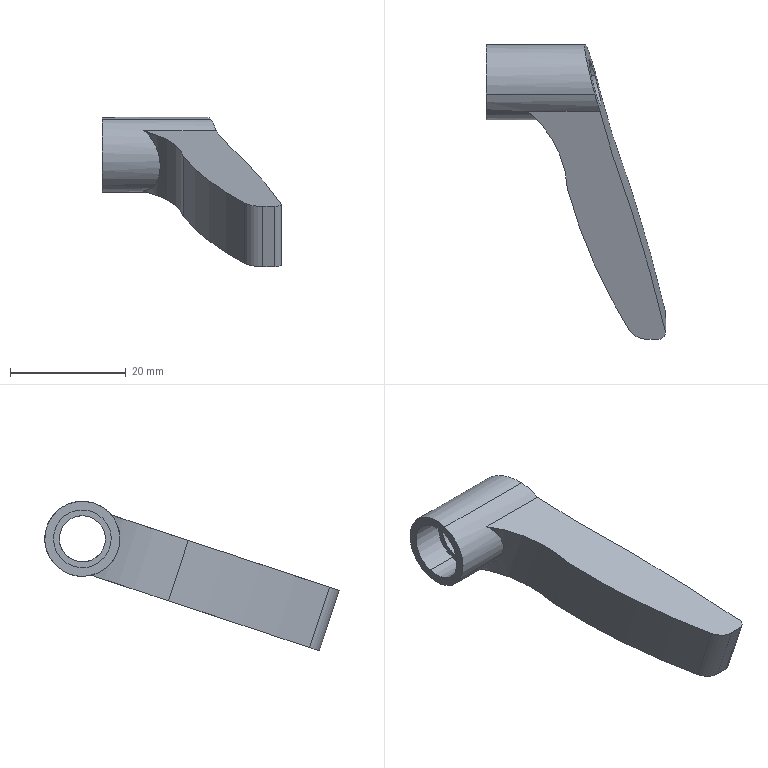Component | SolidWorks | SL010-LeftStreamline-1-1_SL010-2M-0112-000-2-1-1_SL010-CLDM5_25_B-1-1_SL010-_CLDM5_8_B_2_4-1-1 | 1 solid | 17 faces | box 31 x 50.95 x 25.87 mm | volume 5282 mm3 | cylinder 11 | plane 6 | commonest cylinder face diameters 13 x2 10 x2 8 x2 40 x1 200 x1 2.4 x1 600 x1 7.2 x1
STEP:
#1=COLOUR_RGB('',0.7922,0.8196,0.9333);
#2=FILL_AREA_STYLE_COLOUR('',#1);
#3=FILL_AREA_STYLE('',(#2));
#4=SURFACE_STYLE_FILL_AREA(#3);
#5=SURFACE_SIDE_STYLE('',(#4));
#6=SURFACE_STYLE_USAGE(.BOTH.,#5);
#7=PRESENTATION_STYLE_ASSIGNMENT((#6));
#8=CARTESIAN_POINT('',(-5.591,-6.762,-28.28));
#9=VERTEX_POINT('',#8);
#10=CARTESIAN_POINT('',(-5.859,-6.237,-28.106));
#11=VERTEX_POINT('',#10);
#12=CARTESIAN_POINT('',(-6.377,-6.8,-28.293));
#13=DIRECTION('',(0.,-0.3143,0.9493));
#14=DIRECTION('',(0.,-0.9493,-0.3143));
#15=AXIS2_PLACEMENT_3D('',#12,#13,#14);
#16=CIRCLE('',#15,0.7874);
#17=EDGE_CURVE('',#9,#11,#16,.T.);
#18=ORIENTED_EDGE('',*,*,#17,.T.);
#19=CARTESIAN_POINT('',(-5.859,-6.101,-28.518));
#20=VERTEX_POINT('',#19);
#21=CARTESIAN_POINT('',(-5.859,-6.101,-28.518));
#22=CARTESIAN_POINT('',(-5.842,-6.118,-28.513));
#23=CARTESIAN_POINT('',(-5.827,-6.135,-28.507));
#24=CARTESIAN_POINT('',(-5.807,-6.162,-28.494));
#25=CARTESIAN_POINT('',(-5.8,-6.171,-28.489));
#26=CARTESIAN_POINT('',(-5.788,-6.188,-28.478));
#27=CARTESIAN_POINT('',(-5.783,-6.197,-28.471));
#28=CARTESIAN_POINT('',(-5.773,-6.213,-28.457));
#29=CARTESIAN_POINT('',(-5.769,-6.221,-28.449));
#30=CARTESIAN_POINT('',(-5.761,-6.237,-28.432));
#31=CARTESIAN_POINT('',(-5.758,-6.244,-28.423));
#32=CARTESIAN_POINT('',(-5.753,-6.257,-28.404));
#33=CARTESIAN_POINT('',(-5.751,-6.263,-28.394));
#34=CARTESIAN_POINT('',(-5.749,-6.274,-28.372));
#35=CARTESIAN_POINT('',(-5.748,-6.279,-28.361));
#36=CARTESIAN_POINT('',(-5.748,-6.286,-28.339));
#37=CARTESIAN_POINT('',(-5.749,-6.289,-28.327));
#38=CARTESIAN_POINT('',(-5.751,-6.293,-28.303));
#39=CARTESIAN_POINT('',(-5.753,-6.295,-28.291));
#40=CARTESIAN_POINT('',(-5.758,-6.296,-28.268));
#41=CARTESIAN_POINT('',(-5.761,-6.295,-28.256));
#42=CARTESIAN_POINT('',(-5.769,-6.293,-28.234));
#43=CARTESIAN_POINT('',(-5.773,-6.291,-28.222));
#44=CARTESIAN_POINT('',(-5.783,-6.286,-28.201));
#45=CARTESIAN_POINT('',(-5.788,-6.283,-28.191));
#46=CARTESIAN_POINT('',(-5.8,-6.276,-28.171));
#47=CARTESIAN_POINT('',(-5.806,-6.272,-28.162));
#48=CARTESIAN_POINT('',(-5.827,-6.259,-28.135));
#49=CARTESIAN_POINT('',(-5.842,-6.248,-28.12));
#50=CARTESIAN_POINT('',(-5.859,-6.237,-28.106));
#51=B_SPLINE_CURVE_WITH_KNOTS('',3,(#21,#22,#23,#24,#25,#26,#27,#28,#29,#30,#31,#32,#33,#34,#35,#36,#37,#38,#39,#40,#41,#42,#43,#44,#45,#46,#47,#48,#49,#50),.UNSPECIFIED.,.F.,.F.,(4,2,2,2,2,2,2,2,2,2,2,2,2,2,4),(0.,0.00182,0.002729,0.003639,0.004549,0.005459,0.006368,0.007278,0.008188,0.009098,0.01001,0.01092,0.01183,0.01274,0.01456),.UNSPECIFIED.);
#52=EDGE_CURVE('',#20,#11,#51,.T.);
#53=ORIENTED_EDGE('',*,*,#52,.F.);
#54=CARTESIAN_POINT('',(-5.591,-6.626,-28.691));
#55=VERTEX_POINT('',#54);
#56=CARTESIAN_POINT('',(-6.377,-6.664,-28.704));
#57=DIRECTION('',(0.,-0.3143,0.9493));
#58=DIRECTION('',(0.,-0.9493,-0.3143));
#59=AXIS2_PLACEMENT_3D('',#56,#57,#58);
#60=CIRCLE('',#59,0.7874);
#61=EDGE_CURVE('',#55,#20,#60,.T.);
#62=ORIENTED_EDGE('',*,*,#61,.F.);
#63=CARTESIAN_POINT('',(-5.591,-6.762,-28.28));
#64=DIRECTION('',(-0.,0.3143,-0.9493));
#65=VECTOR('',#64,39.37);
#66=LINE('',#63,#65);
#67=EDGE_CURVE('',#9,#55,#66,.T.);
#68=ORIENTED_EDGE('',*,*,#67,.F.);
#69=EDGE_LOOP('',(#18,#53,#62,#68));
#70=FACE_OUTER_BOUND('',#69,.T.);
#71=CARTESIAN_POINT('',(-6.377,-6.8,-28.293));
#72=DIRECTION('',(0.,-0.3143,0.9493));
#73=DIRECTION('',(-0.8993,-0.4152,-0.1375));
#74=AXIS2_PLACEMENT_3D('',#71,#72,#73);
#75=CYLINDRICAL_SURFACE('',#74,0.7874);
#76=ADVANCED_FACE('',(#70),#75,.F.);
#77=CARTESIAN_POINT('',(-5.172,-7.587,-29.01));
#78=VERTEX_POINT('',#77);
#79=CARTESIAN_POINT('',(-1.778,-5.693,-28.382));
#80=DIRECTION('',(0.,-0.3143,0.9493));
#81=DIRECTION('',(0.,-0.9493,-0.3143));
#82=AXIS2_PLACEMENT_3D('',#79,#80,#81);
#83=CIRCLE('',#82,3.937);
#84=EDGE_CURVE('',#55,#78,#83,.T.);
#85=ORIENTED_EDGE('',*,*,#84,.T.);
#86=CARTESIAN_POINT('',(-5.172,-7.723,-28.598));
#87=VERTEX_POINT('',#86);
#88=CARTESIAN_POINT('',(-5.172,-7.723,-28.598));
#89=DIRECTION('',(-0.,0.3143,-0.9493));
#90=VECTOR('',#89,39.37);
#91=LINE('',#88,#90);
#92=EDGE_CURVE('',#87,#78,#91,.T.);
#93=ORIENTED_EDGE('',*,*,#92,.F.);
#94=CARTESIAN_POINT('',(-1.778,-5.829,-27.971));
#95=DIRECTION('',(0.,-0.3143,0.9493));
#96=DIRECTION('',(0.,-0.9493,-0.3143));
#97=AXIS2_PLACEMENT_3D('',#94,#95,#96);
#98=CIRCLE('',#97,3.937);
#99=EDGE_CURVE('',#9,#87,#98,.T.);
#100=ORIENTED_EDGE('',*,*,#99,.F.);
#101=ORIENTED_EDGE('',*,*,#67,.T.);
#102=EDGE_LOOP('',(#85,#93,#100,#101));
#103=FACE_OUTER_BOUND('',#102,.T.);
#104=CARTESIAN_POINT('',(-1.778,-5.829,-27.971));
#105=DIRECTION('',(0.,-0.3143,0.9493));
#106=DIRECTION('',(0.9242,0.3626,0.12));
#107=AXIS2_PLACEMENT_3D('',#104,#105,#106);
#108=CYLINDRICAL_SURFACE('',#107,3.937);
#109=ADVANCED_FACE('',(#103),#108,.T.);
#110=CARTESIAN_POINT('',(-4.921,-7.745,-28.606));
#111=VERTEX_POINT('',#110);
#112=CARTESIAN_POINT('',(-5.287,-6.522,-28.201));
#113=VERTEX_POINT('',#112);
#114=CARTESIAN_POINT('',(-16.448,-10.191,-29.416));
#115=DIRECTION('',(0.,-0.3143,0.9493));
#116=DIRECTION('',(0.,-0.9493,-0.3143));
#117=AXIS2_PLACEMENT_3D('',#114,#115,#116);
#118=CIRCLE('',#117,11.811);
#119=EDGE_CURVE('',#111,#113,#118,.T.);
#120=ORIENTED_EDGE('',*,*,#119,.T.);
#121=CARTESIAN_POINT('',(-5.367,-6.237,-28.106));
#122=VERTEX_POINT('',#121);
#123=CARTESIAN_POINT('',(-5.287,-6.523,-28.201));
#124=DIRECTION('',(-0.2588,0.917,0.3036));
#125=VECTOR('',#124,39.37);
#126=LINE('',#123,#125);
#127=EDGE_CURVE('',#113,#122,#126,.T.);
#128=ORIENTED_EDGE('',*,*,#127,.T.);
#129=CARTESIAN_POINT('',(-6.142,-6.237,-28.106));
#130=DIRECTION('',(-1.,-0.,0.));
#131=VECTOR('',#130,39.37);
#132=LINE('',#129,#131);
#133=EDGE_CURVE('',#122,#11,#132,.T.);
#134=ORIENTED_EDGE('',*,*,#133,.T.);
#135=ORIENTED_EDGE('',*,*,#17,.F.);
#136=ORIENTED_EDGE('',*,*,#99,.T.);
#137=CARTESIAN_POINT('',(-5.05,-7.789,-28.62));
#138=VERTEX_POINT('',#137);
#139=CARTESIAN_POINT('',(-5.05,-7.655,-28.576));
#140=DIRECTION('',(0.,-0.3143,0.9493));
#141=DIRECTION('',(0.,-0.9493,-0.3143));
#142=AXIS2_PLACEMENT_3D('',#139,#140,#141);
#143=CIRCLE('',#142,0.1417);
#144=EDGE_CURVE('',#87,#138,#143,.T.);
#145=ORIENTED_EDGE('',*,*,#144,.T.);
#146=CARTESIAN_POINT('',(-4.969,-7.789,-28.62));
#147=VERTEX_POINT('',#146);
#148=CARTESIAN_POINT('',(-5.05,-7.789,-28.62));
#149=DIRECTION('',(1.,0.,-0.));
#150=VECTOR('',#149,39.37);
#151=LINE('',#148,#150);
#152=EDGE_CURVE('',#138,#147,#151,.T.);
#153=ORIENTED_EDGE('',*,*,#152,.T.);
#154=CARTESIAN_POINT('',(-4.969,-7.745,-28.606));
#155=DIRECTION('',(0.,-0.3143,0.9493));
#156=DIRECTION('',(0.,-0.9493,-0.3143));
#157=AXIS2_PLACEMENT_3D('',#154,#155,#156);
#158=CIRCLE('',#157,0.04724);
#159=EDGE_CURVE('',#147,#111,#158,.T.);
#160=ORIENTED_EDGE('',*,*,#159,.T.);
#161=EDGE_LOOP('',(#120,#128,#134,#135,#136,#145,#153,#160));
#162=FACE_OUTER_BOUND('',#161,.T.);
#163=CARTESIAN_POINT('',(-6.377,-6.8,-28.293));
#164=DIRECTION('',(0.,-0.3143,0.9493));
#165=DIRECTION('',(0.,-0.9493,-0.3143));
#166=AXIS2_PLACEMENT_3D('',#163,#164,#165);
#167=PLANE('',#166);
#168=ADVANCED_FACE('',(#162),#167,.T.);
#169=ORIENTED_EDGE('',*,*,#159,.F.);
#170=CARTESIAN_POINT('',(-4.969,-7.653,-29.032));
#171=VERTEX_POINT('',#170);
#172=CARTESIAN_POINT('',(-4.969,-7.814,-28.546));
#173=DIRECTION('',(-0.,0.3143,-0.9493));
#174=VECTOR('',#173,39.37);
#175=LINE('',#172,#174);
#176=EDGE_CURVE('',#147,#171,#175,.T.);
#177=ORIENTED_EDGE('',*,*,#176,.T.);
#178=CARTESIAN_POINT('',(-4.921,-7.608,-29.017));
#179=VERTEX_POINT('',#178);
#180=CARTESIAN_POINT('',(-4.969,-7.608,-29.017));
#181=DIRECTION('',(0.,-0.3143,0.9493));
#182=DIRECTION('',(0.,-0.9493,-0.3143));
#183=AXIS2_PLACEMENT_3D('',#180,#181,#182);
#184=CIRCLE('',#183,0.04724);
#185=EDGE_CURVE('',#171,#179,#184,.T.);
#186=ORIENTED_EDGE('',*,*,#185,.T.);
#187=CARTESIAN_POINT('',(-4.921,-7.769,-28.531));
#188=DIRECTION('',(-0.,0.3143,-0.9493));
#189=VECTOR('',#188,39.37);
#190=LINE('',#187,#189);
#191=EDGE_CURVE('',#111,#179,#190,.T.);
#192=ORIENTED_EDGE('',*,*,#191,.F.);
#193=EDGE_LOOP('',(#169,#177,#186,#192));
#194=FACE_OUTER_BOUND('',#193,.T.);
#195=CARTESIAN_POINT('',(-4.969,-7.769,-28.531));
#196=DIRECTION('',(0.,-0.3143,0.9493));
#197=DIRECTION('',(-0.7071,0.6713,0.2223));
#198=AXIS2_PLACEMENT_3D('',#195,#196,#197);
#199=CYLINDRICAL_SURFACE('',#198,0.04724);
#200=ADVANCED_FACE('',(#194),#199,.T.);
#201=ORIENTED_EDGE('',*,*,#119,.F.);
#202=ORIENTED_EDGE('',*,*,#191,.T.);
#203=CARTESIAN_POINT('',(-5.287,-6.386,-28.612));
#204=VERTEX_POINT('',#203);
#205=CARTESIAN_POINT('',(-16.448,-10.055,-29.827));
#206=DIRECTION('',(0.,-0.3143,0.9493));
#207=DIRECTION('',(0.,-0.9493,-0.3143));
#208=AXIS2_PLACEMENT_3D('',#205,#206,#207);
#209=CIRCLE('',#208,11.811);
#210=EDGE_CURVE('',#179,#204,#209,.T.);
#211=ORIENTED_EDGE('',*,*,#210,.T.);
#212=CARTESIAN_POINT('',(-5.287,-6.547,-28.126));
#213=DIRECTION('',(-0.,0.3143,-0.9493));
#214=VECTOR('',#213,39.37);
#215=LINE('',#212,#214);
#216=EDGE_CURVE('',#113,#204,#215,.T.);
#217=ORIENTED_EDGE('',*,*,#216,.F.);
#218=EDGE_LOOP('',(#201,#202,#211,#217));
#219=FACE_OUTER_BOUND('',#218,.T.);
#220=CARTESIAN_POINT('',(-16.448,-10.216,-29.341));
#221=DIRECTION('',(0.,-0.3143,0.9493));
#222=DIRECTION('',(-0.962,-0.2593,-0.08585));
#223=AXIS2_PLACEMENT_3D('',#220,#221,#222);
#224=CYLINDRICAL_SURFACE('',#223,11.811);
#225=ADVANCED_FACE('',(#219),#224,.T.);
#226=CARTESIAN_POINT('',(-5.362,-6.189,-28.319));
#227=VERTEX_POINT('',#226);
#228=CARTESIAN_POINT('',(-5.404,-5.99,-28.419));
#229=VERTEX_POINT('',#228);
#230=CARTESIAN_POINT('',(-5.362,-6.189,-28.319));
#231=CARTESIAN_POINT('',(-5.362,-6.183,-28.338));
#232=CARTESIAN_POINT('',(-5.363,-6.172,-28.356));
#233=CARTESIAN_POINT('',(-5.367,-6.145,-28.388));
#234=CARTESIAN_POINT('',(-5.37,-6.129,-28.401));
#235=CARTESIAN_POINT('',(-5.378,-6.092,-28.419));
#236=CARTESIAN_POINT('',(-5.383,-6.072,-28.425));
#237=CARTESIAN_POINT('',(-5.393,-6.03,-28.428));
#238=CARTESIAN_POINT('',(-5.398,-6.01,-28.425));
#239=CARTESIAN_POINT('',(-5.404,-5.99,-28.419));
#240=B_SPLINE_CURVE_WITH_KNOTS('',3,(#230,#231,#232,#233,#234,#235,#236,#237,#238,#239),.UNSPECIFIED.,.F.,.F.,(4,2,2,2,4),(0.,0.3927,0.7854,1.178,1.571),.UNSPECIFIED.);
#241=EDGE_CURVE('',#227,#229,#240,.T.);
#242=ORIENTED_EDGE('',*,*,#241,.F.);
#243=CARTESIAN_POINT('',(-5.404,-6.089,-28.12));
#244=VERTEX_POINT('',#243);
#245=CARTESIAN_POINT('',(-5.404,-6.089,-28.12));
#246=CARTESIAN_POINT('',(-5.398,-6.109,-28.126));
#247=CARTESIAN_POINT('',(-5.393,-6.127,-28.136));
#248=CARTESIAN_POINT('',(-5.383,-6.158,-28.163));
#249=CARTESIAN_POINT('',(-5.378,-6.171,-28.18));
#250=CARTESIAN_POINT('',(-5.37,-6.19,-28.217));
#251=CARTESIAN_POINT('',(-5.367,-6.195,-28.237));
#252=CARTESIAN_POINT('',(-5.363,-6.198,-28.278));
#253=CARTESIAN_POINT('',(-5.362,-6.196,-28.299));
#254=CARTESIAN_POINT('',(-5.362,-6.189,-28.319));
#255=B_SPLINE_CURVE_WITH_KNOTS('',3,(#245,#246,#247,#248,#249,#250,#251,#252,#253,#254),.UNSPECIFIED.,.F.,.F.,(4,2,2,2,4),(4.712,5.105,5.498,5.89,6.283),.UNSPECIFIED.);
#256=EDGE_CURVE('',#244,#227,#255,.T.);
#257=ORIENTED_EDGE('',*,*,#256,.F.);
#258=CARTESIAN_POINT('',(-5.404,-5.99,-28.419));
#259=CARTESIAN_POINT('',(-5.409,-5.97,-28.412));
#260=CARTESIAN_POINT('',(-5.415,-5.952,-28.402));
#261=CARTESIAN_POINT('',(-5.425,-5.921,-28.375));
#262=CARTESIAN_POINT('',(-5.43,-5.908,-28.358));
#263=CARTESIAN_POINT('',(-5.438,-5.89,-28.321));
#264=CARTESIAN_POINT('',(-5.441,-5.884,-28.301));
#265=CARTESIAN_POINT('',(-5.445,-5.881,-28.26));
#266=CARTESIAN_POINT('',(-5.446,-5.884,-28.239));
#267=CARTESIAN_POINT('',(-5.446,-5.897,-28.2));
#268=CARTESIAN_POINT('',(-5.445,-5.907,-28.182));
#269=CARTESIAN_POINT('',(-5.441,-5.934,-28.151));
#270=CARTESIAN_POINT('',(-5.438,-5.95,-28.138));
#271=CARTESIAN_POINT('',(-5.43,-5.987,-28.119));
#272=CARTESIAN_POINT('',(-5.425,-6.007,-28.114));
#273=CARTESIAN_POINT('',(-5.415,-6.049,-28.111));
#274=CARTESIAN_POINT('',(-5.409,-6.069,-28.113));
#275=CARTESIAN_POINT('',(-5.404,-6.089,-28.12));
#276=B_SPLINE_CURVE_WITH_KNOTS('',3,(#258,#259,#260,#261,#262,#263,#264,#265,#266,#267,#268,#269,#270,#271,#272,#273,#274,#275),.UNSPECIFIED.,.F.,.F.,(4,2,2,2,2,2,2,2,4),(1.571,1.963,2.356,2.749,3.142,3.534,3.927,4.32,4.712),.UNSPECIFIED.);
#277=EDGE_CURVE('',#229,#244,#276,.T.);
#278=ORIENTED_EDGE('',*,*,#277,.F.);
#279=EDGE_LOOP('',(#242,#257,#278));
#280=FACE_BOUND('',#279,.T.);
#281=ORIENTED_EDGE('',*,*,#216,.T.);
#282=CARTESIAN_POINT('',(-5.367,-6.101,-28.518));
#283=VERTEX_POINT('',#282);
#284=CARTESIAN_POINT('',(-5.287,-6.387,-28.612));
#285=DIRECTION('',(-0.2588,0.917,0.3036));
#286=VECTOR('',#285,39.37);
#287=LINE('',#284,#286);
#288=EDGE_CURVE('',#204,#283,#287,.T.);
#289=ORIENTED_EDGE('',*,*,#288,.T.);
#290=CARTESIAN_POINT('',(-5.404,-5.959,-28.512));
#291=VERTEX_POINT('',#290);
#292=CARTESIAN_POINT('',(-5.367,-6.101,-28.518));
#293=CARTESIAN_POINT('',(-5.373,-6.078,-28.523));
#294=CARTESIAN_POINT('',(-5.379,-6.054,-28.526));
#295=CARTESIAN_POINT('',(-5.391,-6.006,-28.524));
#296=CARTESIAN_POINT('',(-5.398,-5.982,-28.519));
#297=CARTESIAN_POINT('',(-5.404,-5.959,-28.512));
#298=B_SPLINE_CURVE_WITH_KNOTS('',3,(#292,#293,#294,#295,#296,#297),.UNSPECIFIED.,.F.,.F.,(4,2,4),(0.,1.5,3.),.UNSPECIFIED.);
#299=EDGE_CURVE('',#283,#291,#298,.T.);
#300=ORIENTED_EDGE('',*,*,#299,.T.);
#301=CARTESIAN_POINT('',(-5.404,-6.12,-28.026));
#302=VERTEX_POINT('',#301);
#303=CARTESIAN_POINT('',(-5.404,-5.959,-28.512));
#304=CARTESIAN_POINT('',(-5.408,-5.945,-28.507));
#305=CARTESIAN_POINT('',(-5.412,-5.93,-28.501));
#306=CARTESIAN_POINT('',(-5.421,-5.902,-28.486));
#307=CARTESIAN_POINT('',(-5.425,-5.888,-28.476));
#308=CARTESIAN_POINT('',(-5.433,-5.862,-28.455));
#309=CARTESIAN_POINT('',(-5.437,-5.85,-28.442));
#310=CARTESIAN_POINT('',(-5.445,-5.828,-28.415));
#311=CARTESIAN_POINT('',(-5.449,-5.819,-28.4));
#312=CARTESIAN_POINT('',(-5.456,-5.803,-28.368));
#313=CARTESIAN_POINT('',(-5.459,-5.797,-28.352));
#314=CARTESIAN_POINT('',(-5.464,-5.788,-28.318));
#315=CARTESIAN_POINT('',(-5.466,-5.785,-28.301));
#316=CARTESIAN_POINT('',(-5.469,-5.783,-28.267));
#317=CARTESIAN_POINT('',(-5.471,-5.784,-28.25));
#318=CARTESIAN_POINT('',(-5.472,-5.788,-28.218));
#319=CARTESIAN_POINT('',(-5.472,-5.792,-28.203));
#320=CARTESIAN_POINT('',(-5.472,-5.801,-28.174));
#321=CARTESIAN_POINT('',(-5.472,-5.808,-28.16));
#322=CARTESIAN_POINT('',(-5.471,-5.823,-28.132));
#323=CARTESIAN_POINT('',(-5.469,-5.832,-28.118));
#324=CARTESIAN_POINT('',(-5.466,-5.854,-28.092));
#325=CARTESIAN_POINT('',(-5.464,-5.867,-28.08));
#326=CARTESIAN_POINT('',(-5.459,-5.894,-28.058));
#327=CARTESIAN_POINT('',(-5.456,-5.909,-28.048));
#328=CARTESIAN_POINT('',(-5.449,-5.94,-28.033));
#329=CARTESIAN_POINT('',(-5.445,-5.957,-28.026));
#330=CARTESIAN_POINT('',(-5.437,-5.991,-28.017));
#331=CARTESIAN_POINT('',(-5.433,-6.008,-28.015));
#332=CARTESIAN_POINT('',(-5.425,-6.042,-28.013));
#333=CARTESIAN_POINT('',(-5.421,-6.058,-28.013));
#334=CARTESIAN_POINT('',(-5.412,-6.09,-28.018));
#335=CARTESIAN_POINT('',(-5.408,-6.106,-28.021));
#336=CARTESIAN_POINT('',(-5.404,-6.12,-28.026));
#337=B_SPLINE_CURVE_WITH_KNOTS('',3,(#303,#304,#305,#306,#307,#308,#309,#310,#311,#312,#313,#314,#315,#316,#317,#318,#319,#320,#321,#322,#323,#324,#325,#326,#327,#328,#329,#330,#331,#332,#333,#334,#335,#336),.UNSPECIFIED.,.F.,.F.,(4,2,2,2,2,2,2,2,2,2,2,2,2,2,2,2,4),(0.,0.0625,0.125,0.1875,0.25,0.3125,0.375,0.4375,0.5,0.5625,0.625,0.6875,0.75,0.8125,0.875,0.9375,1.),.UNSPECIFIED.);
#338=EDGE_CURVE('',#291,#302,#337,.T.);
#339=ORIENTED_EDGE('',*,*,#338,.T.);
#340=CARTESIAN_POINT('',(-5.404,-6.12,-28.026));
#341=CARTESIAN_POINT('',(-5.398,-6.142,-28.034));
#342=CARTESIAN_POINT('',(-5.391,-6.164,-28.044));
#343=CARTESIAN_POINT('',(-5.379,-6.204,-28.072));
#344=CARTESIAN_POINT('',(-5.373,-6.222,-28.088));
#345=CARTESIAN_POINT('',(-5.367,-6.237,-28.106));
#346=B_SPLINE_CURVE_WITH_KNOTS('',3,(#340,#341,#342,#343,#344,#345),.UNSPECIFIED.,.F.,.F.,(4,2,4),(0.,1.5,3.),.UNSPECIFIED.);
#347=EDGE_CURVE('',#302,#122,#346,.T.);
#348=ORIENTED_EDGE('',*,*,#347,.T.);
#349=ORIENTED_EDGE('',*,*,#127,.F.);
#350=EDGE_LOOP('',(#281,#289,#300,#339,#348,#349));
#351=FACE_OUTER_BOUND('',#350,.T.);
#352=CARTESIAN_POINT('',(-5.472,-5.889,-27.908));
#353=DIRECTION('',(0.9659,0.2457,0.08135));
#354=DIRECTION('',(-0.2588,0.917,0.3036));
#355=AXIS2_PLACEMENT_3D('',#352,#353,#354);
#356=PLANE('',#355);
#357=ADVANCED_FACE('',(#280,#351),#356,.T.);
#358=CARTESIAN_POINT('',(-6.142,-5.959,-28.512));
#359=VERTEX_POINT('',#358);
#360=CARTESIAN_POINT('',(-6.142,-6.12,-28.026));
#361=VERTEX_POINT('',#360);
#362=CARTESIAN_POINT('',(-6.142,-6.04,-28.269));
#363=DIRECTION('',(-1.,-0.,0.));
#364=DIRECTION('',(0.,0.3143,-0.9493));
#365=AXIS2_PLACEMENT_3D('',#362,#363,#364);
#366=CIRCLE('',#365,0.2559);
#367=EDGE_CURVE('',#359,#361,#366,.T.);
#368=ORIENTED_EDGE('',*,*,#367,.F.);
#369=CARTESIAN_POINT('',(-6.142,-5.959,-28.512));
#370=DIRECTION('',(1.,0.,-0.));
#371=VECTOR('',#370,39.37);
#372=LINE('',#369,#371);
#373=EDGE_CURVE('',#359,#291,#372,.T.);
#374=ORIENTED_EDGE('',*,*,#373,.T.);
#375=ORIENTED_EDGE('',*,*,#299,.F.);
#376=CARTESIAN_POINT('',(-6.142,-6.101,-28.518));
#377=DIRECTION('',(-1.,-0.,0.));
#378=VECTOR('',#377,39.37);
#379=LINE('',#376,#378);
#380=EDGE_CURVE('',#283,#20,#379,.T.);
#381=ORIENTED_EDGE('',*,*,#380,.T.);
#382=ORIENTED_EDGE('',*,*,#52,.T.);
#383=ORIENTED_EDGE('',*,*,#133,.F.);
#384=ORIENTED_EDGE('',*,*,#347,.F.);
#385=CARTESIAN_POINT('',(-6.142,-6.12,-28.026));
#386=DIRECTION('',(1.,0.,-0.));
#387=VECTOR('',#386,39.37);
#388=LINE('',#385,#387);
#389=EDGE_CURVE('',#361,#302,#388,.T.);
#390=ORIENTED_EDGE('',*,*,#389,.F.);
#391=EDGE_LOOP('',(#368,#374,#375,#381,#382,#383,#384,#390));
#392=FACE_OUTER_BOUND('',#391,.T.);
#393=CARTESIAN_POINT('',(-6.142,-6.04,-28.269));
#394=DIRECTION('',(1.,0.,-0.));
#395=DIRECTION('',(0.,0.9493,0.3143));
#396=AXIS2_PLACEMENT_3D('',#393,#394,#395);
#397=CYLINDRICAL_SURFACE('',#396,0.2559);
#398=ADVANCED_FACE('',(#392),#397,.T.);
#399=ORIENTED_EDGE('',*,*,#338,.F.);
#400=ORIENTED_EDGE('',*,*,#373,.F.);
#401=CARTESIAN_POINT('',(-6.142,-6.04,-28.269));
#402=DIRECTION('',(-1.,-0.,0.));
#403=DIRECTION('',(0.,0.3143,-0.9493));
#404=AXIS2_PLACEMENT_3D('',#401,#402,#403);
#405=CIRCLE('',#404,0.2559);
#406=EDGE_CURVE('',#361,#359,#405,.T.);
#407=ORIENTED_EDGE('',*,*,#406,.F.);
#408=ORIENTED_EDGE('',*,*,#389,.T.);
#409=EDGE_LOOP('',(#399,#400,#407,#408));
#410=FACE_OUTER_BOUND('',#409,.T.);
#411=CARTESIAN_POINT('',(-6.142,-6.04,-28.269));
#412=DIRECTION('',(1.,0.,-0.));
#413=DIRECTION('',(0.,-0.9493,-0.3143));
#414=AXIS2_PLACEMENT_3D('',#411,#412,#413);
#415=CYLINDRICAL_SURFACE('',#414,0.2559);
#416=ADVANCED_FACE('',(#410),#415,.T.);
#417=CARTESIAN_POINT('',(-6.142,-6.101,-28.082));
#418=VERTEX_POINT('',#417);
#419=CARTESIAN_POINT('',(-6.142,-5.978,-28.456));
#420=VERTEX_POINT('',#419);
#421=CARTESIAN_POINT('',(-6.142,-6.04,-28.269));
#422=DIRECTION('',(1.,0.,-0.));
#423=DIRECTION('',(0.,-0.3143,0.9493));
#424=AXIS2_PLACEMENT_3D('',#421,#422,#423);
#425=CIRCLE('',#424,0.1969);
#426=EDGE_CURVE('',#418,#420,#425,.T.);
#427=ORIENTED_EDGE('',*,*,#426,.T.);
#428=CARTESIAN_POINT('',(-6.142,-6.04,-28.269));
#429=DIRECTION('',(1.,0.,-0.));
#430=DIRECTION('',(0.,-0.3143,0.9493));
#431=AXIS2_PLACEMENT_3D('',#428,#429,#430);
#432=CIRCLE('',#431,0.1969);
#433=EDGE_CURVE('',#420,#418,#432,.T.);
#434=ORIENTED_EDGE('',*,*,#433,.T.);
#435=EDGE_LOOP('',(#427,#434));
#436=FACE_BOUND('',#435,.T.);
#437=ORIENTED_EDGE('',*,*,#367,.T.);
#438=ORIENTED_EDGE('',*,*,#406,.T.);
#439=EDGE_LOOP('',(#437,#438));
#440=FACE_OUTER_BOUND('',#439,.T.);
#441=CARTESIAN_POINT('',(-6.142,-6.282,-28.35));
#442=DIRECTION('',(1.,0.,-0.));
#443=DIRECTION('',(0.,-0.3143,0.9493));
#444=AXIS2_PLACEMENT_3D('',#441,#442,#443);
#445=PLANE('',#444);
#446=ADVANCED_FACE('',(#436,#440),#445,.F.);
#447=ORIENTED_EDGE('',*,*,#433,.F.);
#448=CARTESIAN_POINT('',(-5.929,-5.978,-28.456));
#449=VERTEX_POINT('',#448);
#450=CARTESIAN_POINT('',(-5.929,-5.978,-28.456));
#451=DIRECTION('',(-1.,-0.,0.));
#452=VECTOR('',#451,39.37);
#453=LINE('',#450,#452);
#454=EDGE_CURVE('',#449,#420,#453,.T.);
#455=ORIENTED_EDGE('',*,*,#454,.F.);
#456=CARTESIAN_POINT('',(-5.929,-6.101,-28.082));
#457=VERTEX_POINT('',#456);
#458=CARTESIAN_POINT('',(-5.929,-6.04,-28.269));
#459=DIRECTION('',(1.,0.,-0.));
#460=DIRECTION('',(0.,-0.3143,0.9493));
#461=AXIS2_PLACEMENT_3D('',#458,#459,#460);
#462=CIRCLE('',#461,0.1969);
#463=EDGE_CURVE('',#449,#457,#462,.T.);
#464=ORIENTED_EDGE('',*,*,#463,.T.);
#465=CARTESIAN_POINT('',(-5.929,-6.101,-28.082));
#466=DIRECTION('',(-1.,-0.,0.));
#467=VECTOR('',#466,39.37);
#468=LINE('',#465,#467);
#469=EDGE_CURVE('',#457,#418,#468,.T.);
#470=ORIENTED_EDGE('',*,*,#469,.T.);
#471=EDGE_LOOP('',(#447,#455,#464,#470));
#472=FACE_OUTER_BOUND('',#471,.T.);
#473=CARTESIAN_POINT('',(-4.331,-6.04,-28.269));
#474=DIRECTION('',(-1.,-0.,0.));
#475=DIRECTION('',(0.,-0.9493,-0.3143));
#476=AXIS2_PLACEMENT_3D('',#473,#474,#475);
#477=CYLINDRICAL_SURFACE('',#476,0.1969);
#478=ADVANCED_FACE('',(#472),#477,.F.);
#479=CARTESIAN_POINT('',(-5.929,-6.04,-28.269));
#480=DIRECTION('',(1.,0.,-0.));
#481=DIRECTION('',(0.,-0.3143,0.9493));
#482=AXIS2_PLACEMENT_3D('',#479,#480,#481);
#483=CIRCLE('',#482,0.1969);
#484=EDGE_CURVE('',#457,#449,#483,.T.);
#485=ORIENTED_EDGE('',*,*,#484,.T.);
#486=ORIENTED_EDGE('',*,*,#454,.T.);
#487=ORIENTED_EDGE('',*,*,#426,.F.);
#488=ORIENTED_EDGE('',*,*,#469,.F.);
#489=EDGE_LOOP('',(#485,#486,#487,#488));
#490=FACE_OUTER_BOUND('',#489,.T.);
#491=CARTESIAN_POINT('',(-4.331,-6.04,-28.269));
#492=DIRECTION('',(-1.,-0.,0.));
#493=DIRECTION('',(0.,0.9493,0.3143));
#494=AXIS2_PLACEMENT_3D('',#491,#492,#493);
#495=CYLINDRICAL_SURFACE('',#494,0.1969);
#496=ADVANCED_FACE('',(#490),#495,.F.);
#497=CARTESIAN_POINT('',(-5.929,-6.089,-28.12));
#498=VERTEX_POINT('',#497);
#499=CARTESIAN_POINT('',(-5.929,-5.99,-28.419));
#500=VERTEX_POINT('',#499);
#501=CARTESIAN_POINT('',(-5.929,-6.04,-28.269));
#502=DIRECTION('',(1.,0.,-0.));
#503=DIRECTION('',(0.,-0.3143,0.9493));
#504=AXIS2_PLACEMENT_3D('',#501,#502,#503);
#505=CIRCLE('',#504,0.1575);
#506=EDGE_CURVE('',#498,#500,#505,.T.);
#507=ORIENTED_EDGE('',*,*,#506,.T.);
#508=CARTESIAN_POINT('',(-5.929,-6.04,-28.269));
#509=DIRECTION('',(1.,0.,-0.));
#510=DIRECTION('',(0.,-0.3143,0.9493));
#511=AXIS2_PLACEMENT_3D('',#508,#509,#510);
#512=CIRCLE('',#511,0.1575);
#513=EDGE_CURVE('',#500,#498,#512,.T.);
#514=ORIENTED_EDGE('',*,*,#513,.T.);
#515=EDGE_LOOP('',(#507,#514));
#516=FACE_BOUND('',#515,.T.);
#517=ORIENTED_EDGE('',*,*,#484,.F.);
#518=ORIENTED_EDGE('',*,*,#463,.F.);
#519=EDGE_LOOP('',(#517,#518));
#520=FACE_OUTER_BOUND('',#519,.T.);
#521=CARTESIAN_POINT('',(-5.929,-5.853,-28.207));
#522=DIRECTION('',(-1.,-0.,0.));
#523=DIRECTION('',(-0.,0.3143,-0.9493));
#524=AXIS2_PLACEMENT_3D('',#521,#522,#523);
#525=PLANE('',#524);
#526=ADVANCED_FACE('',(#516,#520),#525,.T.);
#527=ORIENTED_EDGE('',*,*,#513,.F.);
#528=CARTESIAN_POINT('',(-5.404,-5.99,-28.419));
#529=DIRECTION('',(-1.,-0.,0.));
#530=VECTOR('',#529,39.37);
#531=LINE('',#528,#530);
#532=EDGE_CURVE('',#229,#500,#531,.T.);
#533=ORIENTED_EDGE('',*,*,#532,.F.);
#534=ORIENTED_EDGE('',*,*,#277,.T.);
#535=CARTESIAN_POINT('',(-5.404,-6.089,-28.12));
#536=DIRECTION('',(-1.,-0.,0.));
#537=VECTOR('',#536,39.37);
#538=LINE('',#535,#537);
#539=EDGE_CURVE('',#244,#498,#538,.T.);
#540=ORIENTED_EDGE('',*,*,#539,.T.);
#541=EDGE_LOOP('',(#527,#533,#534,#540));
#542=FACE_OUTER_BOUND('',#541,.T.);
#543=CARTESIAN_POINT('',(-4.331,-6.04,-28.269));
#544=DIRECTION('',(-1.,-0.,0.));
#545=DIRECTION('',(0.,-0.9493,-0.3143));
#546=AXIS2_PLACEMENT_3D('',#543,#544,#545);
#547=CYLINDRICAL_SURFACE('',#546,0.1575);
#548=ADVANCED_FACE('',(#542),#547,.F.);
#549=ORIENTED_EDGE('',*,*,#241,.T.);
#550=ORIENTED_EDGE('',*,*,#532,.T.);
#551=ORIENTED_EDGE('',*,*,#506,.F.);
#552=ORIENTED_EDGE('',*,*,#539,.F.);
#553=ORIENTED_EDGE('',*,*,#256,.T.);
#554=EDGE_LOOP('',(#549,#550,#551,#552,#553));
#555=FACE_OUTER_BOUND('',#554,.T.);
#556=CARTESIAN_POINT('',(-4.331,-6.04,-28.269));
#557=DIRECTION('',(-1.,-0.,0.));
#558=DIRECTION('',(0.,0.9493,0.3143));
#559=AXIS2_PLACEMENT_3D('',#556,#557,#558);
#560=CYLINDRICAL_SURFACE('',#559,0.1575);
#561=ADVANCED_FACE('',(#555),#560,.F.);
#562=ORIENTED_EDGE('',*,*,#288,.F.);
#563=ORIENTED_EDGE('',*,*,#210,.F.);
#564=ORIENTED_EDGE('',*,*,#185,.F.);
#565=CARTESIAN_POINT('',(-5.05,-7.653,-29.032));
#566=VERTEX_POINT('',#565);
#567=CARTESIAN_POINT('',(-5.05,-7.653,-29.032));
#568=DIRECTION('',(1.,0.,-0.));
#569=VECTOR('',#568,39.37);
#570=LINE('',#567,#569);
#571=EDGE_CURVE('',#566,#171,#570,.T.);
#572=ORIENTED_EDGE('',*,*,#571,.F.);
#573=CARTESIAN_POINT('',(-5.05,-7.519,-28.987));
#574=DIRECTION('',(0.,-0.3143,0.9493));
#575=DIRECTION('',(0.,-0.9493,-0.3143));
#576=AXIS2_PLACEMENT_3D('',#573,#574,#575);
#577=CIRCLE('',#576,0.1417);
#578=EDGE_CURVE('',#78,#566,#577,.T.);
#579=ORIENTED_EDGE('',*,*,#578,.F.);
#580=ORIENTED_EDGE('',*,*,#84,.F.);
#581=ORIENTED_EDGE('',*,*,#61,.T.);
#582=ORIENTED_EDGE('',*,*,#380,.F.);
#583=EDGE_LOOP('',(#562,#563,#564,#572,#579,#580,#581,#582));
#584=FACE_OUTER_BOUND('',#583,.T.);
#585=CARTESIAN_POINT('',(-6.377,-6.664,-28.704));
#586=DIRECTION('',(0.,-0.3143,0.9493));
#587=DIRECTION('',(0.,-0.9493,-0.3143));
#588=AXIS2_PLACEMENT_3D('',#585,#586,#587);
#589=PLANE('',#588);
#590=ADVANCED_FACE('',(#584),#589,.F.);
#591=ORIENTED_EDGE('',*,*,#578,.T.);
#592=CARTESIAN_POINT('',(-5.05,-7.789,-28.62));
#593=DIRECTION('',(-0.,0.3143,-0.9493));
#594=VECTOR('',#593,39.37);
#595=LINE('',#592,#594);
#596=EDGE_CURVE('',#138,#566,#595,.T.);
#597=ORIENTED_EDGE('',*,*,#596,.F.);
#598=ORIENTED_EDGE('',*,*,#144,.F.);
#599=ORIENTED_EDGE('',*,*,#92,.T.);
#600=EDGE_LOOP('',(#591,#597,#598,#599));
#601=FACE_OUTER_BOUND('',#600,.T.);
#602=CARTESIAN_POINT('',(-5.05,-7.655,-28.576));
#603=DIRECTION('',(0.,-0.3143,0.9493));
#604=DIRECTION('',(0.4966,0.824,0.2728));
#605=AXIS2_PLACEMENT_3D('',#602,#603,#604);
#606=CYLINDRICAL_SURFACE('',#605,0.1417);
#607=ADVANCED_FACE('',(#601),#606,.T.);
#608=ORIENTED_EDGE('',*,*,#571,.T.);
#609=ORIENTED_EDGE('',*,*,#176,.F.);
#610=ORIENTED_EDGE('',*,*,#152,.F.);
#611=ORIENTED_EDGE('',*,*,#596,.T.);
#612=EDGE_LOOP('',(#608,#609,#610,#611));
#613=FACE_OUTER_BOUND('',#612,.T.);
#614=CARTESIAN_POINT('',(-5.05,-7.789,-28.62));
#615=DIRECTION('',(0.,0.9493,0.3143));
#616=DIRECTION('',(0.,-0.3143,0.9493));
#617=AXIS2_PLACEMENT_3D('',#614,#615,#616);
#618=PLANE('',#617);
#619=ADVANCED_FACE('',(#613),#618,.F.);
#620=CLOSED_SHELL('',(#76,#109,#168,#200,#225,#357,#398,#416,#446,#478,#496,#526,#548,#561,#590,#607,#619));
#621=MANIFOLD_SOLID_BREP('',#620);
#622=STYLED_ITEM('',(#7),#621);
#623=PRESENTATION_LAYER_ASSIGNMENT('','',(#622));
#624=CARTESIAN_POINT('',(0.,0.,0.));
#625=DIRECTION('',(0.,0.,1.));
#626=DIRECTION('',(1.,0.,0.));
#627=AXIS2_PLACEMENT_3D('',#624,#625,#626);
#628=(LENGTH_UNIT()NAMED_UNIT(*)SI_UNIT($,.METRE.));
#629=LENGTH_MEASURE_WITH_UNIT(LENGTH_MEASURE(0.0254),#628);
#630=DIMENSIONAL_EXPONENTS(1.,0.,0.,0.,0.,0.,0.);
#631=(CONVERSION_BASED_UNIT('',#629)LENGTH_UNIT()NAMED_UNIT(#630));
#632=UNCERTAINTY_MEASURE_WITH_UNIT(LENGTH_MEASURE(0.00001),#631,'','');
#633=(NAMED_UNIT(*)PLANE_ANGLE_UNIT()SI_UNIT($,.RADIAN.));
#634=(NAMED_UNIT(*)SI_UNIT($,.STERADIAN.)SOLID_ANGLE_UNIT());
#635=(GEOMETRIC_REPRESENTATION_CONTEXT(3)GLOBAL_UNCERTAINTY_ASSIGNED_CONTEXT((#632))GLOBAL_UNIT_ASSIGNED_CONTEXT((#631,#633,#634))REPRESENTATION_CONTEXT('',''));
#636=ADVANCED_BREP_SHAPE_REPRESENTATION('',(#621,#627),#635);
#637=(LENGTH_UNIT()NAMED_UNIT(*)SI_UNIT($,.METRE.));
#638=LENGTH_MEASURE_WITH_UNIT(LENGTH_MEASURE(0.0254),#637);
#639=DIMENSIONAL_EXPONENTS(1.,0.,0.,0.,0.,0.,0.);
#640=(CONVERSION_BASED_UNIT('',#638)LENGTH_UNIT()NAMED_UNIT(#639));
#641=UNCERTAINTY_MEASURE_WITH_UNIT(LENGTH_MEASURE(0.00001),#640,'','');
#642=(NAMED_UNIT(*)PLANE_ANGLE_UNIT()SI_UNIT($,.RADIAN.));
#643=(NAMED_UNIT(*)SI_UNIT($,.STERADIAN.)SOLID_ANGLE_UNIT());
#644=(GEOMETRIC_REPRESENTATION_CONTEXT(3)GLOBAL_UNCERTAINTY_ASSIGNED_CONTEXT((#641))GLOBAL_UNIT_ASSIGNED_CONTEXT((#640,#642,#643))REPRESENTATION_CONTEXT('',''));
#645=MECHANICAL_DESIGN_GEOMETRIC_PRESENTATION_REPRESENTATION('',(#622),#644);